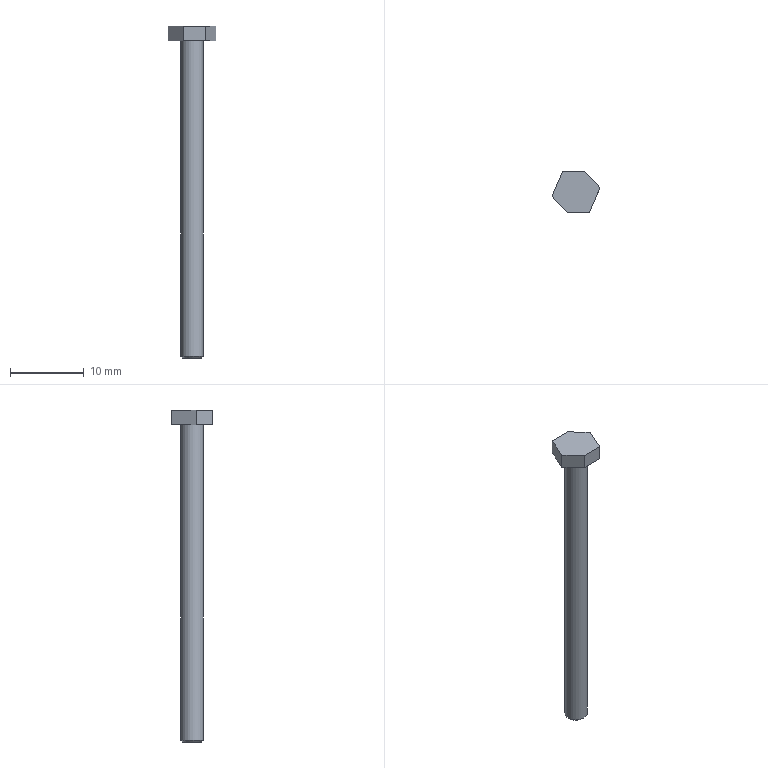Component | NX | LONG_SCREW_M3_2 | 1 solid | 11 faces | box 6.48 x 5.5 x 45 mm | volume 356 mm3 | plane 9 | cylinder 1 | cone 1 | commonest cylinder face diameters 3 x1
STEP:
#1=CARTESIAN_POINT('',(0.,0.,0.));
#2=DIRECTION('',(0.,0.,1.));
#3=DIRECTION('',(1.,0.,0.));
#4=AXIS2_PLACEMENT_3D('',#1,#2,#3);
#5=CARTESIAN_POINT('',(-13.131,-4.443,15.25));
#6=VERTEX_POINT('',#5);
#7=CARTESIAN_POINT('',(-14.506,-3.843,15.25));
#8=DIRECTION('',(0.,0.,1.));
#9=DIRECTION('',(0.9167,-0.3997,0.));
#10=AXIS2_PLACEMENT_3D('',#7,#8,#9);
#11=CIRCLE('',#10,1.5);
#12=CARTESIAN_POINT('',(-14.506,-3.843,15.));
#13=DIRECTION('',(0.,0.,1.));
#14=DIRECTION('',(0.9167,-0.3997,0.));
#15=AXIS2_PLACEMENT_3D('',#12,#13,#14);
#16=CYLINDRICAL_SURFACE('',#15,1.5);
#17=CARTESIAN_POINT('',(0.,0.25));
#18=DIRECTION('',(1.,0.));
#19=VECTOR('',#18,1.);
#20=LINE('',#17,#19);
#21=(GEOMETRIC_REPRESENTATION_CONTEXT(2)PARAMETRIC_REPRESENTATION_CONTEXT()REPRESENTATION_CONTEXT('',''));
#22=DEFINITIONAL_REPRESENTATION('',(#20),#21);
#23=PCURVE('',#16,#22);
#24=CARTESIAN_POINT('',(-14.506,-3.843,15.25));
#25=DIRECTION('',(0.,0.,1.));
#26=DIRECTION('',(0.9167,-0.3997,0.));
#27=AXIS2_PLACEMENT_3D('',#24,#25,#26);
#28=CONICAL_SURFACE('',#27,1.5,0.7854);
#29=CARTESIAN_POINT('',(0.,0.));
#30=DIRECTION('',(1.,0.));
#31=VECTOR('',#30,1.);
#32=LINE('',#29,#31);
#33=(GEOMETRIC_REPRESENTATION_CONTEXT(2)PARAMETRIC_REPRESENTATION_CONTEXT()REPRESENTATION_CONTEXT('',''));
#34=DEFINITIONAL_REPRESENTATION('',(#32),#33);
#35=PCURVE('',#28,#34);
#36=SURFACE_CURVE('',#11,(#23,#35),.PCURVE_S1.);
#37=EDGE_CURVE('',#6,#6,#36,.T.);
#38=ORIENTED_EDGE('',*,*,#37,.T.);
#39=CARTESIAN_POINT('',(-13.131,-4.443,58.));
#40=VERTEX_POINT('',#39);
#41=CARTESIAN_POINT('',(-13.131,-4.443,15.25));
#42=CARTESIAN_POINT('',(-13.131,-4.443,58.));
#43=B_SPLINE_CURVE_WITH_KNOTS('',1,(#41,#42),.UNSPECIFIED.,.F.,.F.,(2,2),(0.25,43.),.PIECEWISE_BEZIER_KNOTS.);
#44=CARTESIAN_POINT('',(6.283,0.));
#45=DIRECTION('',(0.,1.));
#46=VECTOR('',#45,1.);
#47=LINE('',#44,#46);
#48=(GEOMETRIC_REPRESENTATION_CONTEXT(2)PARAMETRIC_REPRESENTATION_CONTEXT()REPRESENTATION_CONTEXT('',''));
#49=DEFINITIONAL_REPRESENTATION('',(#47),#48);
#50=PCURVE('',#16,#49);
#51=CARTESIAN_POINT('',(0.,0.));
#52=DIRECTION('',(0.,1.));
#53=VECTOR('',#52,1.);
#54=LINE('',#51,#53);
#55=(GEOMETRIC_REPRESENTATION_CONTEXT(2)PARAMETRIC_REPRESENTATION_CONTEXT()REPRESENTATION_CONTEXT('',''));
#56=DEFINITIONAL_REPRESENTATION('',(#54),#55);
#57=PCURVE('',#16,#56);
#58=SEAM_CURVE('',#43,(#50,#57),.PCURVE_S1.);
#59=EDGE_CURVE('',#6,#40,#58,.T.);
#60=ORIENTED_EDGE('',*,*,#59,.T.);
#61=CARTESIAN_POINT('',(-14.506,-3.843,58.));
#62=DIRECTION('',(0.,0.,1.));
#63=DIRECTION('',(0.9167,-0.3997,0.));
#64=AXIS2_PLACEMENT_3D('',#61,#62,#63);
#65=CIRCLE('',#64,1.5);
#66=CARTESIAN_POINT('',(0.,43.));
#67=DIRECTION('',(1.,0.));
#68=VECTOR('',#67,1.);
#69=LINE('',#66,#68);
#70=(GEOMETRIC_REPRESENTATION_CONTEXT(2)PARAMETRIC_REPRESENTATION_CONTEXT()REPRESENTATION_CONTEXT('',''));
#71=DEFINITIONAL_REPRESENTATION('',(#69),#70);
#72=PCURVE('',#16,#71);
#73=CARTESIAN_POINT('',(-17.746,-4.395,58.));
#74=DIRECTION('',(0.,0.,1.));
#75=DIRECTION('',(0.9167,-0.3997,0.));
#76=AXIS2_PLACEMENT_3D('',#73,#74,#75);
#77=PLANE('',#76);
#78=CARTESIAN_POINT('',(2.75,1.801));
#79=DIRECTION('',(1.,-0.));
#80=AXIS2_PLACEMENT_2D('',#78,#79);
#81=CIRCLE('',#80,1.5);
#82=(GEOMETRIC_REPRESENTATION_CONTEXT(2)PARAMETRIC_REPRESENTATION_CONTEXT()REPRESENTATION_CONTEXT('',''));
#83=DEFINITIONAL_REPRESENTATION('',(#81),#82);
#84=PCURVE('',#77,#83);
#85=SURFACE_CURVE('',#65,(#72,#84),.PCURVE_S1.);
#86=EDGE_CURVE('',#40,#40,#85,.T.);
#87=ORIENTED_EDGE('',*,*,#86,.F.);
#88=ORIENTED_EDGE('',*,*,#59,.F.);
#89=EDGE_LOOP('',(#38,#60,#87,#88));
#90=FACE_BOUND('',#89,.T.);
#91=ADVANCED_FACE('',(#90),#16,.T.);
#92=CARTESIAN_POINT('',(-13.36,-4.343,15.));
#93=VERTEX_POINT('',#92);
#94=CARTESIAN_POINT('',(-14.506,-3.843,15.));
#95=DIRECTION('',(0.,0.,-1.));
#96=DIRECTION('',(0.9167,-0.3997,0.));
#97=AXIS2_PLACEMENT_3D('',#94,#95,#96);
#98=CIRCLE('',#97,1.25);
#99=CARTESIAN_POINT('',(-14.506,-3.843,15.));
#100=DIRECTION('',(0.,0.,1.));
#101=DIRECTION('',(0.9167,-0.3997,0.));
#102=AXIS2_PLACEMENT_3D('',#99,#100,#101);
#103=PLANE('',#102);
#104=CARTESIAN_POINT('',(1.25,0.));
#105=CARTESIAN_POINT('',(1.25,-2.165));
#106=CARTESIAN_POINT('',(-0.625,-1.083));
#107=CARTESIAN_POINT('',(-2.5,-0.));
#108=CARTESIAN_POINT('',(-0.625,1.083));
#109=CARTESIAN_POINT('',(1.25,2.165));
#110=CARTESIAN_POINT('',(1.25,0.));
#111=(BOUNDED_CURVE()B_SPLINE_CURVE(2,(#104,#105,#106,#107,#108,#109,#110),.UNSPECIFIED.,.T.,.F.)B_SPLINE_CURVE_WITH_KNOTS((1,2,2,2,2,1),(-2.094,0.,2.094,4.189,6.283,8.378),.UNSPECIFIED.)CURVE()GEOMETRIC_REPRESENTATION_ITEM()RATIONAL_B_SPLINE_CURVE((1.,0.5,1.,0.5,1.,0.5,1.))REPRESENTATION_ITEM(''));
#112=(GEOMETRIC_REPRESENTATION_CONTEXT(2)PARAMETRIC_REPRESENTATION_CONTEXT()REPRESENTATION_CONTEXT('',''));
#113=DEFINITIONAL_REPRESENTATION('',(#111),#112);
#114=PCURVE('',#103,#113);
#115=CARTESIAN_POINT('',(6.283,-0.25));
#116=DIRECTION('',(-1.,0.));
#117=VECTOR('',#116,1.);
#118=LINE('',#115,#117);
#119=(GEOMETRIC_REPRESENTATION_CONTEXT(2)PARAMETRIC_REPRESENTATION_CONTEXT()REPRESENTATION_CONTEXT('',''));
#120=DEFINITIONAL_REPRESENTATION('',(#118),#119);
#121=PCURVE('',#28,#120);
#122=SURFACE_CURVE('',#98,(#114,#121),.PCURVE_S1.);
#123=EDGE_CURVE('',#93,#93,#122,.T.);
#124=ORIENTED_EDGE('',*,*,#123,.T.);
#125=EDGE_LOOP('',(#124));
#126=FACE_BOUND('',#125,.T.);
#127=ADVANCED_FACE('',(#126),#103,.F.);
#128=CARTESIAN_POINT('',(-17.746,-4.395,58.));
#129=VERTEX_POINT('',#128);
#130=CARTESIAN_POINT('',(-15.705,-6.593,58.));
#131=VERTEX_POINT('',#130);
#132=CARTESIAN_POINT('',(-17.746,-4.395,58.));
#133=DIRECTION('',(0.6806,-0.7327,0.));
#134=VECTOR('',#133,1.);
#135=LINE('',#132,#134);
#136=CARTESIAN_POINT('',(0.,0.));
#137=DIRECTION('',(0.9167,-0.3997));
#138=VECTOR('',#137,1.);
#139=LINE('',#136,#138);
#140=(GEOMETRIC_REPRESENTATION_CONTEXT(2)PARAMETRIC_REPRESENTATION_CONTEXT()REPRESENTATION_CONTEXT('',''));
#141=DEFINITIONAL_REPRESENTATION('',(#139),#140);
#142=PCURVE('',#77,#141);
#143=CARTESIAN_POINT('',(-17.746,-4.395,60.));
#144=DIRECTION('',(0.7327,0.6806,0.));
#145=DIRECTION('',(-0.6806,0.7327,0.));
#146=AXIS2_PLACEMENT_3D('',#143,#144,#145);
#147=PLANE('',#146);
#148=CARTESIAN_POINT('',(0.,-2.));
#149=DIRECTION('',(-1.,0.));
#150=VECTOR('',#149,1.);
#151=LINE('',#148,#150);
#152=(GEOMETRIC_REPRESENTATION_CONTEXT(2)PARAMETRIC_REPRESENTATION_CONTEXT()REPRESENTATION_CONTEXT('',''));
#153=DEFINITIONAL_REPRESENTATION('',(#151),#152);
#154=PCURVE('',#147,#153);
#155=SURFACE_CURVE('',#135,(#142,#154),.PCURVE_S1.);
#156=EDGE_CURVE('',#129,#131,#155,.T.);
#157=ORIENTED_EDGE('',*,*,#156,.F.);
#158=CARTESIAN_POINT('',(-16.307,-1.093,58.));
#159=VERTEX_POINT('',#158);
#160=CARTESIAN_POINT('',(-16.307,-1.093,58.));
#161=DIRECTION('',(-0.3997,-0.9167,0.));
#162=VECTOR('',#161,1.);
#163=LINE('',#160,#162);
#164=CARTESIAN_POINT('',(0.,3.602));
#165=DIRECTION('',(-0.,-1.));
#166=VECTOR('',#165,1.);
#167=LINE('',#164,#166);
#168=(GEOMETRIC_REPRESENTATION_CONTEXT(2)PARAMETRIC_REPRESENTATION_CONTEXT()REPRESENTATION_CONTEXT('',''));
#169=DEFINITIONAL_REPRESENTATION('',(#167),#168);
#170=PCURVE('',#77,#169);
#171=CARTESIAN_POINT('',(-16.307,-1.093,60.));
#172=DIRECTION('',(0.9167,-0.3997,0.));
#173=DIRECTION('',(0.3997,0.9167,0.));
#174=AXIS2_PLACEMENT_3D('',#171,#172,#173);
#175=PLANE('',#174);
#176=CARTESIAN_POINT('',(0.,-2.));
#177=DIRECTION('',(-1.,0.));
#178=VECTOR('',#177,1.);
#179=LINE('',#176,#178);
#180=(GEOMETRIC_REPRESENTATION_CONTEXT(2)PARAMETRIC_REPRESENTATION_CONTEXT()REPRESENTATION_CONTEXT('',''));
#181=DEFINITIONAL_REPRESENTATION('',(#179),#180);
#182=PCURVE('',#175,#181);
#183=SURFACE_CURVE('',#163,(#170,#182),.PCURVE_S1.);
#184=EDGE_CURVE('',#159,#129,#183,.T.);
#185=ORIENTED_EDGE('',*,*,#184,.F.);
#186=CARTESIAN_POINT('',(-13.307,-1.093,58.));
#187=VERTEX_POINT('',#186);
#188=CARTESIAN_POINT('',(-13.307,-1.093,58.));
#189=DIRECTION('',(-1.,0.,0.));
#190=VECTOR('',#189,1.);
#191=LINE('',#188,#190);
#192=CARTESIAN_POINT('',(2.75,4.801));
#193=DIRECTION('',(-0.9167,-0.3997));
#194=VECTOR('',#193,1.);
#195=LINE('',#192,#194);
#196=(GEOMETRIC_REPRESENTATION_CONTEXT(2)PARAMETRIC_REPRESENTATION_CONTEXT()REPRESENTATION_CONTEXT('',''));
#197=DEFINITIONAL_REPRESENTATION('',(#195),#196);
#198=PCURVE('',#77,#197);
#199=CARTESIAN_POINT('',(-13.307,-1.093,60.));
#200=DIRECTION('',(-0.,-1.,0.));
#201=DIRECTION('',(1.,-0.,0.));
#202=AXIS2_PLACEMENT_3D('',#199,#200,#201);
#203=PLANE('',#202);
#204=CARTESIAN_POINT('',(0.,-2.));
#205=DIRECTION('',(-1.,0.));
#206=VECTOR('',#205,1.);
#207=LINE('',#204,#206);
#208=(GEOMETRIC_REPRESENTATION_CONTEXT(2)PARAMETRIC_REPRESENTATION_CONTEXT()REPRESENTATION_CONTEXT('',''));
#209=DEFINITIONAL_REPRESENTATION('',(#207),#208);
#210=PCURVE('',#203,#209);
#211=SURFACE_CURVE('',#191,(#198,#210),.PCURVE_S1.);
#212=EDGE_CURVE('',#187,#159,#211,.T.);
#213=ORIENTED_EDGE('',*,*,#212,.F.);
#214=CARTESIAN_POINT('',(-11.265,-3.291,58.));
#215=VERTEX_POINT('',#214);
#216=CARTESIAN_POINT('',(-11.265,-3.291,58.));
#217=DIRECTION('',(-0.6806,0.7327,0.));
#218=VECTOR('',#217,1.);
#219=LINE('',#216,#218);
#220=CARTESIAN_POINT('',(5.5,3.602));
#221=DIRECTION('',(-0.9167,0.3997));
#222=VECTOR('',#221,1.);
#223=LINE('',#220,#222);
#224=(GEOMETRIC_REPRESENTATION_CONTEXT(2)PARAMETRIC_REPRESENTATION_CONTEXT()REPRESENTATION_CONTEXT('',''));
#225=DEFINITIONAL_REPRESENTATION('',(#223),#224);
#226=PCURVE('',#77,#225);
#227=CARTESIAN_POINT('',(-11.265,-3.291,60.));
#228=DIRECTION('',(-0.7327,-0.6806,0.));
#229=DIRECTION('',(0.6806,-0.7327,0.));
#230=AXIS2_PLACEMENT_3D('',#227,#228,#229);
#231=PLANE('',#230);
#232=CARTESIAN_POINT('',(0.,-2.));
#233=DIRECTION('',(-1.,0.));
#234=VECTOR('',#233,1.);
#235=LINE('',#232,#234);
#236=(GEOMETRIC_REPRESENTATION_CONTEXT(2)PARAMETRIC_REPRESENTATION_CONTEXT()REPRESENTATION_CONTEXT('',''));
#237=DEFINITIONAL_REPRESENTATION('',(#235),#236);
#238=PCURVE('',#231,#237);
#239=SURFACE_CURVE('',#219,(#226,#238),.PCURVE_S1.);
#240=EDGE_CURVE('',#215,#187,#239,.T.);
#241=ORIENTED_EDGE('',*,*,#240,.F.);
#242=CARTESIAN_POINT('',(-12.705,-6.593,58.));
#243=VERTEX_POINT('',#242);
#244=CARTESIAN_POINT('',(-11.985,-4.942,58.));
#245=DIRECTION('',(0.3997,0.9167,0.));
#246=VECTOR('',#245,1.);
#247=LINE('',#244,#246);
#248=CARTESIAN_POINT('',(5.5,1.801));
#249=DIRECTION('',(0.,1.));
#250=VECTOR('',#249,1.);
#251=LINE('',#248,#250);
#252=(GEOMETRIC_REPRESENTATION_CONTEXT(2)PARAMETRIC_REPRESENTATION_CONTEXT()REPRESENTATION_CONTEXT('',''));
#253=DEFINITIONAL_REPRESENTATION('',(#251),#252);
#254=PCURVE('',#77,#253);
#255=CARTESIAN_POINT('',(-11.985,-4.942,60.));
#256=DIRECTION('',(-0.9167,0.3997,0.));
#257=DIRECTION('',(0.,0.,1.));
#258=AXIS2_PLACEMENT_3D('',#255,#256,#257);
#259=PLANE('',#258);
#260=CARTESIAN_POINT('',(-2.,0.));
#261=DIRECTION('',(0.,1.));
#262=VECTOR('',#261,1.);
#263=LINE('',#260,#262);
#264=(GEOMETRIC_REPRESENTATION_CONTEXT(2)PARAMETRIC_REPRESENTATION_CONTEXT()REPRESENTATION_CONTEXT('',''));
#265=DEFINITIONAL_REPRESENTATION('',(#263),#264);
#266=PCURVE('',#259,#265);
#267=SURFACE_CURVE('',#247,(#254,#266),.PCURVE_S1.);
#268=EDGE_CURVE('',#243,#215,#267,.T.);
#269=ORIENTED_EDGE('',*,*,#268,.F.);
#270=CARTESIAN_POINT('',(-15.705,-6.593,58.));
#271=DIRECTION('',(1.,0.,0.));
#272=VECTOR('',#271,1.);
#273=LINE('',#270,#272);
#274=CARTESIAN_POINT('',(2.75,-1.199));
#275=DIRECTION('',(0.9167,0.3997));
#276=VECTOR('',#275,1.);
#277=LINE('',#274,#276);
#278=(GEOMETRIC_REPRESENTATION_CONTEXT(2)PARAMETRIC_REPRESENTATION_CONTEXT()REPRESENTATION_CONTEXT('',''));
#279=DEFINITIONAL_REPRESENTATION('',(#277),#278);
#280=PCURVE('',#77,#279);
#281=CARTESIAN_POINT('',(-15.705,-6.593,60.));
#282=DIRECTION('',(0.,1.,0.));
#283=DIRECTION('',(-1.,0.,0.));
#284=AXIS2_PLACEMENT_3D('',#281,#282,#283);
#285=PLANE('',#284);
#286=CARTESIAN_POINT('',(0.,-2.));
#287=DIRECTION('',(-1.,0.));
#288=VECTOR('',#287,1.);
#289=LINE('',#286,#288);
#290=(GEOMETRIC_REPRESENTATION_CONTEXT(2)PARAMETRIC_REPRESENTATION_CONTEXT()REPRESENTATION_CONTEXT('',''));
#291=DEFINITIONAL_REPRESENTATION('',(#289),#290);
#292=PCURVE('',#285,#291);
#293=SURFACE_CURVE('',#273,(#280,#292),.PCURVE_S1.);
#294=EDGE_CURVE('',#131,#243,#293,.T.);
#295=ORIENTED_EDGE('',*,*,#294,.F.);
#296=EDGE_LOOP('',(#157,#185,#213,#241,#269,#295));
#297=FACE_BOUND('',#296,.T.);
#298=ORIENTED_EDGE('',*,*,#86,.T.);
#299=EDGE_LOOP('',(#298));
#300=FACE_BOUND('',#299,.T.);
#301=ADVANCED_FACE('',(#297,#300),#77,.F.);
#302=ORIENTED_EDGE('',*,*,#156,.T.);
#303=CARTESIAN_POINT('',(-15.705,-6.593,60.));
#304=VERTEX_POINT('',#303);
#305=CARTESIAN_POINT('',(-15.705,-6.593,60.));
#306=DIRECTION('',(0.,0.,-1.));
#307=VECTOR('',#306,1.);
#308=LINE('',#305,#307);
#309=CARTESIAN_POINT('',(-3.,0.));
#310=DIRECTION('',(0.,-1.));
#311=VECTOR('',#310,1.);
#312=LINE('',#309,#311);
#313=(GEOMETRIC_REPRESENTATION_CONTEXT(2)PARAMETRIC_REPRESENTATION_CONTEXT()REPRESENTATION_CONTEXT('',''));
#314=DEFINITIONAL_REPRESENTATION('',(#312),#313);
#315=PCURVE('',#147,#314);
#316=CARTESIAN_POINT('',(0.,0.));
#317=DIRECTION('',(0.,-1.));
#318=VECTOR('',#317,1.);
#319=LINE('',#316,#318);
#320=(GEOMETRIC_REPRESENTATION_CONTEXT(2)PARAMETRIC_REPRESENTATION_CONTEXT()REPRESENTATION_CONTEXT('',''));
#321=DEFINITIONAL_REPRESENTATION('',(#319),#320);
#322=PCURVE('',#285,#321);
#323=SURFACE_CURVE('',#308,(#315,#322),.PCURVE_S1.);
#324=EDGE_CURVE('',#304,#131,#323,.T.);
#325=ORIENTED_EDGE('',*,*,#324,.F.);
#326=CARTESIAN_POINT('',(-17.746,-4.395,60.));
#327=VERTEX_POINT('',#326);
#328=CARTESIAN_POINT('',(-17.746,-4.395,60.));
#329=DIRECTION('',(0.6806,-0.7327,0.));
#330=VECTOR('',#329,1.);
#331=LINE('',#328,#330);
#332=CARTESIAN_POINT('',(0.,0.));
#333=DIRECTION('',(-1.,0.));
#334=VECTOR('',#333,1.);
#335=LINE('',#332,#334);
#336=(GEOMETRIC_REPRESENTATION_CONTEXT(2)PARAMETRIC_REPRESENTATION_CONTEXT()REPRESENTATION_CONTEXT('',''));
#337=DEFINITIONAL_REPRESENTATION('',(#335),#336);
#338=PCURVE('',#147,#337);
#339=CARTESIAN_POINT('',(-17.746,-4.395,60.));
#340=DIRECTION('',(0.,0.,1.));
#341=DIRECTION('',(0.9167,-0.3997,0.));
#342=AXIS2_PLACEMENT_3D('',#339,#340,#341);
#343=PLANE('',#342);
#344=CARTESIAN_POINT('',(0.,0.));
#345=DIRECTION('',(0.9167,-0.3997));
#346=VECTOR('',#345,1.);
#347=LINE('',#344,#346);
#348=(GEOMETRIC_REPRESENTATION_CONTEXT(2)PARAMETRIC_REPRESENTATION_CONTEXT()REPRESENTATION_CONTEXT('',''));
#349=DEFINITIONAL_REPRESENTATION('',(#347),#348);
#350=PCURVE('',#343,#349);
#351=SURFACE_CURVE('',#331,(#338,#350),.PCURVE_S1.);
#352=EDGE_CURVE('',#327,#304,#351,.T.);
#353=ORIENTED_EDGE('',*,*,#352,.F.);
#354=CARTESIAN_POINT('',(-17.746,-4.395,60.));
#355=DIRECTION('',(0.,0.,-1.));
#356=VECTOR('',#355,1.);
#357=LINE('',#354,#356);
#358=CARTESIAN_POINT('',(0.,0.));
#359=DIRECTION('',(0.,-1.));
#360=VECTOR('',#359,1.);
#361=LINE('',#358,#360);
#362=(GEOMETRIC_REPRESENTATION_CONTEXT(2)PARAMETRIC_REPRESENTATION_CONTEXT()REPRESENTATION_CONTEXT('',''));
#363=DEFINITIONAL_REPRESENTATION('',(#361),#362);
#364=PCURVE('',#147,#363);
#365=CARTESIAN_POINT('',(-3.602,0.));
#366=DIRECTION('',(0.,-1.));
#367=VECTOR('',#366,1.);
#368=LINE('',#365,#367);
#369=(GEOMETRIC_REPRESENTATION_CONTEXT(2)PARAMETRIC_REPRESENTATION_CONTEXT()REPRESENTATION_CONTEXT('',''));
#370=DEFINITIONAL_REPRESENTATION('',(#368),#369);
#371=PCURVE('',#175,#370);
#372=SURFACE_CURVE('',#357,(#364,#371),.PCURVE_S1.);
#373=EDGE_CURVE('',#327,#129,#372,.T.);
#374=ORIENTED_EDGE('',*,*,#373,.T.);
#375=EDGE_LOOP('',(#302,#325,#353,#374));
#376=FACE_BOUND('',#375,.T.);
#377=ADVANCED_FACE('',(#376),#147,.F.);
#378=ORIENTED_EDGE('',*,*,#294,.T.);
#379=CARTESIAN_POINT('',(-12.705,-6.593,60.));
#380=VERTEX_POINT('',#379);
#381=CARTESIAN_POINT('',(-12.705,-6.593,60.));
#382=DIRECTION('',(0.,0.,-1.));
#383=VECTOR('',#382,1.);
#384=LINE('',#381,#383);
#385=CARTESIAN_POINT('',(-3.,0.));
#386=DIRECTION('',(0.,-1.));
#387=VECTOR('',#386,1.);
#388=LINE('',#385,#387);
#389=(GEOMETRIC_REPRESENTATION_CONTEXT(2)PARAMETRIC_REPRESENTATION_CONTEXT()REPRESENTATION_CONTEXT('',''));
#390=DEFINITIONAL_REPRESENTATION('',(#388),#389);
#391=PCURVE('',#285,#390);
#392=CARTESIAN_POINT('',(0.,-1.801));
#393=DIRECTION('',(-1.,0.));
#394=VECTOR('',#393,1.);
#395=LINE('',#392,#394);
#396=(GEOMETRIC_REPRESENTATION_CONTEXT(2)PARAMETRIC_REPRESENTATION_CONTEXT()REPRESENTATION_CONTEXT('',''));
#397=DEFINITIONAL_REPRESENTATION('',(#395),#396);
#398=PCURVE('',#259,#397);
#399=SURFACE_CURVE('',#384,(#391,#398),.PCURVE_S1.);
#400=EDGE_CURVE('',#380,#243,#399,.T.);
#401=ORIENTED_EDGE('',*,*,#400,.F.);
#402=CARTESIAN_POINT('',(-15.705,-6.593,60.));
#403=DIRECTION('',(1.,0.,0.));
#404=VECTOR('',#403,1.);
#405=LINE('',#402,#404);
#406=CARTESIAN_POINT('',(0.,0.));
#407=DIRECTION('',(-1.,0.));
#408=VECTOR('',#407,1.);
#409=LINE('',#406,#408);
#410=(GEOMETRIC_REPRESENTATION_CONTEXT(2)PARAMETRIC_REPRESENTATION_CONTEXT()REPRESENTATION_CONTEXT('',''));
#411=DEFINITIONAL_REPRESENTATION('',(#409),#410);
#412=PCURVE('',#285,#411);
#413=CARTESIAN_POINT('',(2.75,-1.199));
#414=DIRECTION('',(0.9167,0.3997));
#415=VECTOR('',#414,1.);
#416=LINE('',#413,#415);
#417=(GEOMETRIC_REPRESENTATION_CONTEXT(2)PARAMETRIC_REPRESENTATION_CONTEXT()REPRESENTATION_CONTEXT('',''));
#418=DEFINITIONAL_REPRESENTATION('',(#416),#417);
#419=PCURVE('',#343,#418);
#420=SURFACE_CURVE('',#405,(#412,#419),.PCURVE_S1.);
#421=EDGE_CURVE('',#304,#380,#420,.T.);
#422=ORIENTED_EDGE('',*,*,#421,.F.);
#423=ORIENTED_EDGE('',*,*,#324,.T.);
#424=EDGE_LOOP('',(#378,#401,#422,#423));
#425=FACE_BOUND('',#424,.T.);
#426=ADVANCED_FACE('',(#425),#285,.F.);
#427=ORIENTED_EDGE('',*,*,#268,.T.);
#428=CARTESIAN_POINT('',(-11.265,-3.291,60.));
#429=VERTEX_POINT('',#428);
#430=CARTESIAN_POINT('',(-11.265,-3.291,60.));
#431=DIRECTION('',(0.,0.,-1.));
#432=VECTOR('',#431,1.);
#433=LINE('',#430,#432);
#434=CARTESIAN_POINT('',(0.,1.801));
#435=DIRECTION('',(-1.,0.));
#436=VECTOR('',#435,1.);
#437=LINE('',#434,#436);
#438=(GEOMETRIC_REPRESENTATION_CONTEXT(2)PARAMETRIC_REPRESENTATION_CONTEXT()REPRESENTATION_CONTEXT('',''));
#439=DEFINITIONAL_REPRESENTATION('',(#437),#438);
#440=PCURVE('',#259,#439);
#441=CARTESIAN_POINT('',(0.,0.));
#442=DIRECTION('',(0.,-1.));
#443=VECTOR('',#442,1.);
#444=LINE('',#441,#443);
#445=(GEOMETRIC_REPRESENTATION_CONTEXT(2)PARAMETRIC_REPRESENTATION_CONTEXT()REPRESENTATION_CONTEXT('',''));
#446=DEFINITIONAL_REPRESENTATION('',(#444),#445);
#447=PCURVE('',#231,#446);
#448=SURFACE_CURVE('',#433,(#440,#447),.PCURVE_S1.);
#449=EDGE_CURVE('',#429,#215,#448,.T.);
#450=ORIENTED_EDGE('',*,*,#449,.F.);
#451=CARTESIAN_POINT('',(-12.705,-6.593,60.));
#452=DIRECTION('',(0.3997,0.9167,0.));
#453=VECTOR('',#452,1.);
#454=LINE('',#451,#453);
#455=CARTESIAN_POINT('',(0.,-1.801));
#456=DIRECTION('',(0.,1.));
#457=VECTOR('',#456,1.);
#458=LINE('',#455,#457);
#459=(GEOMETRIC_REPRESENTATION_CONTEXT(2)PARAMETRIC_REPRESENTATION_CONTEXT()REPRESENTATION_CONTEXT('',''));
#460=DEFINITIONAL_REPRESENTATION('',(#458),#459);
#461=PCURVE('',#259,#460);
#462=CARTESIAN_POINT('',(5.5,0.));
#463=DIRECTION('',(0.,1.));
#464=VECTOR('',#463,1.);
#465=LINE('',#462,#464);
#466=(GEOMETRIC_REPRESENTATION_CONTEXT(2)PARAMETRIC_REPRESENTATION_CONTEXT()REPRESENTATION_CONTEXT('',''));
#467=DEFINITIONAL_REPRESENTATION('',(#465),#466);
#468=PCURVE('',#343,#467);
#469=SURFACE_CURVE('',#454,(#461,#468),.PCURVE_S1.);
#470=EDGE_CURVE('',#380,#429,#469,.T.);
#471=ORIENTED_EDGE('',*,*,#470,.F.);
#472=ORIENTED_EDGE('',*,*,#400,.T.);
#473=EDGE_LOOP('',(#427,#450,#471,#472));
#474=FACE_BOUND('',#473,.T.);
#475=ADVANCED_FACE('',(#474),#259,.F.);
#476=ORIENTED_EDGE('',*,*,#240,.T.);
#477=CARTESIAN_POINT('',(-13.307,-1.093,60.));
#478=VERTEX_POINT('',#477);
#479=CARTESIAN_POINT('',(-13.307,-1.093,60.));
#480=DIRECTION('',(0.,0.,-1.));
#481=VECTOR('',#480,1.);
#482=LINE('',#479,#481);
#483=CARTESIAN_POINT('',(-3.,0.));
#484=DIRECTION('',(0.,-1.));
#485=VECTOR('',#484,1.);
#486=LINE('',#483,#485);
#487=(GEOMETRIC_REPRESENTATION_CONTEXT(2)PARAMETRIC_REPRESENTATION_CONTEXT()REPRESENTATION_CONTEXT('',''));
#488=DEFINITIONAL_REPRESENTATION('',(#486),#487);
#489=PCURVE('',#231,#488);
#490=CARTESIAN_POINT('',(0.,0.));
#491=DIRECTION('',(0.,-1.));
#492=VECTOR('',#491,1.);
#493=LINE('',#490,#492);
#494=(GEOMETRIC_REPRESENTATION_CONTEXT(2)PARAMETRIC_REPRESENTATION_CONTEXT()REPRESENTATION_CONTEXT('',''));
#495=DEFINITIONAL_REPRESENTATION('',(#493),#494);
#496=PCURVE('',#203,#495);
#497=SURFACE_CURVE('',#482,(#489,#496),.PCURVE_S1.);
#498=EDGE_CURVE('',#478,#187,#497,.T.);
#499=ORIENTED_EDGE('',*,*,#498,.F.);
#500=CARTESIAN_POINT('',(-11.265,-3.291,60.));
#501=DIRECTION('',(-0.6806,0.7327,0.));
#502=VECTOR('',#501,1.);
#503=LINE('',#500,#502);
#504=CARTESIAN_POINT('',(0.,0.));
#505=DIRECTION('',(-1.,0.));
#506=VECTOR('',#505,1.);
#507=LINE('',#504,#506);
#508=(GEOMETRIC_REPRESENTATION_CONTEXT(2)PARAMETRIC_REPRESENTATION_CONTEXT()REPRESENTATION_CONTEXT('',''));
#509=DEFINITIONAL_REPRESENTATION('',(#507),#508);
#510=PCURVE('',#231,#509);
#511=CARTESIAN_POINT('',(5.5,3.602));
#512=DIRECTION('',(-0.9167,0.3997));
#513=VECTOR('',#512,1.);
#514=LINE('',#511,#513);
#515=(GEOMETRIC_REPRESENTATION_CONTEXT(2)PARAMETRIC_REPRESENTATION_CONTEXT()REPRESENTATION_CONTEXT('',''));
#516=DEFINITIONAL_REPRESENTATION('',(#514),#515);
#517=PCURVE('',#343,#516);
#518=SURFACE_CURVE('',#503,(#510,#517),.PCURVE_S1.);
#519=EDGE_CURVE('',#429,#478,#518,.T.);
#520=ORIENTED_EDGE('',*,*,#519,.F.);
#521=ORIENTED_EDGE('',*,*,#449,.T.);
#522=EDGE_LOOP('',(#476,#499,#520,#521));
#523=FACE_BOUND('',#522,.T.);
#524=ADVANCED_FACE('',(#523),#231,.F.);
#525=ORIENTED_EDGE('',*,*,#212,.T.);
#526=CARTESIAN_POINT('',(-16.307,-1.093,60.));
#527=VERTEX_POINT('',#526);
#528=CARTESIAN_POINT('',(-16.307,-1.093,60.));
#529=DIRECTION('',(0.,0.,-1.));
#530=VECTOR('',#529,1.);
#531=LINE('',#528,#530);
#532=CARTESIAN_POINT('',(-3.,0.));
#533=DIRECTION('',(0.,-1.));
#534=VECTOR('',#533,1.);
#535=LINE('',#532,#534);
#536=(GEOMETRIC_REPRESENTATION_CONTEXT(2)PARAMETRIC_REPRESENTATION_CONTEXT()REPRESENTATION_CONTEXT('',''));
#537=DEFINITIONAL_REPRESENTATION('',(#535),#536);
#538=PCURVE('',#203,#537);
#539=CARTESIAN_POINT('',(0.,0.));
#540=DIRECTION('',(0.,-1.));
#541=VECTOR('',#540,1.);
#542=LINE('',#539,#541);
#543=(GEOMETRIC_REPRESENTATION_CONTEXT(2)PARAMETRIC_REPRESENTATION_CONTEXT()REPRESENTATION_CONTEXT('',''));
#544=DEFINITIONAL_REPRESENTATION('',(#542),#543);
#545=PCURVE('',#175,#544);
#546=SURFACE_CURVE('',#531,(#538,#545),.PCURVE_S1.);
#547=EDGE_CURVE('',#527,#159,#546,.T.);
#548=ORIENTED_EDGE('',*,*,#547,.F.);
#549=CARTESIAN_POINT('',(-13.307,-1.093,60.));
#550=DIRECTION('',(-1.,0.,0.));
#551=VECTOR('',#550,1.);
#552=LINE('',#549,#551);
#553=CARTESIAN_POINT('',(0.,0.));
#554=DIRECTION('',(-1.,0.));
#555=VECTOR('',#554,1.);
#556=LINE('',#553,#555);
#557=(GEOMETRIC_REPRESENTATION_CONTEXT(2)PARAMETRIC_REPRESENTATION_CONTEXT()REPRESENTATION_CONTEXT('',''));
#558=DEFINITIONAL_REPRESENTATION('',(#556),#557);
#559=PCURVE('',#203,#558);
#560=CARTESIAN_POINT('',(2.75,4.801));
#561=DIRECTION('',(-0.9167,-0.3997));
#562=VECTOR('',#561,1.);
#563=LINE('',#560,#562);
#564=(GEOMETRIC_REPRESENTATION_CONTEXT(2)PARAMETRIC_REPRESENTATION_CONTEXT()REPRESENTATION_CONTEXT('',''));
#565=DEFINITIONAL_REPRESENTATION('',(#563),#564);
#566=PCURVE('',#343,#565);
#567=SURFACE_CURVE('',#552,(#559,#566),.PCURVE_S1.);
#568=EDGE_CURVE('',#478,#527,#567,.T.);
#569=ORIENTED_EDGE('',*,*,#568,.F.);
#570=ORIENTED_EDGE('',*,*,#498,.T.);
#571=EDGE_LOOP('',(#525,#548,#569,#570));
#572=FACE_BOUND('',#571,.T.);
#573=ADVANCED_FACE('',(#572),#203,.F.);
#574=ORIENTED_EDGE('',*,*,#184,.T.);
#575=ORIENTED_EDGE('',*,*,#373,.F.);
#576=CARTESIAN_POINT('',(-17.026,-2.744,60.));
#577=DIRECTION('',(-0.3997,-0.9167,0.));
#578=VECTOR('',#577,1.);
#579=LINE('',#576,#578);
#580=CARTESIAN_POINT('',(-1.801,0.));
#581=DIRECTION('',(-1.,0.));
#582=VECTOR('',#581,1.);
#583=LINE('',#580,#582);
#584=(GEOMETRIC_REPRESENTATION_CONTEXT(2)PARAMETRIC_REPRESENTATION_CONTEXT()REPRESENTATION_CONTEXT('',''));
#585=DEFINITIONAL_REPRESENTATION('',(#583),#584);
#586=PCURVE('',#175,#585);
#587=CARTESIAN_POINT('',(0.,1.801));
#588=DIRECTION('',(0.,-1.));
#589=VECTOR('',#588,1.);
#590=LINE('',#587,#589);
#591=(GEOMETRIC_REPRESENTATION_CONTEXT(2)PARAMETRIC_REPRESENTATION_CONTEXT()REPRESENTATION_CONTEXT('',''));
#592=DEFINITIONAL_REPRESENTATION('',(#590),#591);
#593=PCURVE('',#343,#592);
#594=SURFACE_CURVE('',#579,(#586,#593),.PCURVE_S1.);
#595=EDGE_CURVE('',#527,#327,#594,.T.);
#596=ORIENTED_EDGE('',*,*,#595,.F.);
#597=ORIENTED_EDGE('',*,*,#547,.T.);
#598=EDGE_LOOP('',(#574,#575,#596,#597));
#599=FACE_BOUND('',#598,.T.);
#600=ADVANCED_FACE('',(#599),#175,.F.);
#601=ORIENTED_EDGE('',*,*,#595,.T.);
#602=ORIENTED_EDGE('',*,*,#352,.T.);
#603=ORIENTED_EDGE('',*,*,#421,.T.);
#604=ORIENTED_EDGE('',*,*,#470,.T.);
#605=ORIENTED_EDGE('',*,*,#519,.T.);
#606=ORIENTED_EDGE('',*,*,#568,.T.);
#607=EDGE_LOOP('',(#601,#602,#603,#604,#605,#606));
#608=FACE_BOUND('',#607,.T.);
#609=ADVANCED_FACE('',(#608),#343,.T.);
#610=ORIENTED_EDGE('',*,*,#123,.F.);
#611=CARTESIAN_POINT('',(-13.36,-4.343,15.));
#612=CARTESIAN_POINT('',(-13.131,-4.443,15.25));
#613=B_SPLINE_CURVE_WITH_KNOTS('',1,(#611,#612),.UNSPECIFIED.,.F.,.F.,(2,2),(-0.3536,0.),.PIECEWISE_BEZIER_KNOTS.);
#614=CARTESIAN_POINT('',(6.283,0.));
#615=DIRECTION('',(0.,1.));
#616=VECTOR('',#615,1.);
#617=LINE('',#614,#616);
#618=(GEOMETRIC_REPRESENTATION_CONTEXT(2)PARAMETRIC_REPRESENTATION_CONTEXT()REPRESENTATION_CONTEXT('',''));
#619=DEFINITIONAL_REPRESENTATION('',(#617),#618);
#620=PCURVE('',#28,#619);
#621=CARTESIAN_POINT('',(0.,0.));
#622=DIRECTION('',(0.,1.));
#623=VECTOR('',#622,1.);
#624=LINE('',#621,#623);
#625=(GEOMETRIC_REPRESENTATION_CONTEXT(2)PARAMETRIC_REPRESENTATION_CONTEXT()REPRESENTATION_CONTEXT('',''));
#626=DEFINITIONAL_REPRESENTATION('',(#624),#625);
#627=PCURVE('',#28,#626);
#628=SEAM_CURVE('',#613,(#620,#627),.PCURVE_S1.);
#629=EDGE_CURVE('',#93,#6,#628,.T.);
#630=ORIENTED_EDGE('',*,*,#629,.T.);
#631=ORIENTED_EDGE('',*,*,#37,.F.);
#632=ORIENTED_EDGE('',*,*,#629,.F.);
#633=EDGE_LOOP('',(#610,#630,#631,#632));
#634=FACE_BOUND('',#633,.T.);
#635=ADVANCED_FACE('',(#634),#28,.T.);
#636=CLOSED_SHELL('',(#91,#127,#301,#377,#426,#475,#524,#573,#600,#609,#635));
#637=MANIFOLD_SOLID_BREP('',#636);
#638=(LENGTH_UNIT()NAMED_UNIT(*)SI_UNIT(.MILLI.,.METRE.));
#639=UNCERTAINTY_MEASURE_WITH_UNIT(LENGTH_MEASURE(0.000002),#638,'','');
#640=(NAMED_UNIT(*)PLANE_ANGLE_UNIT()SI_UNIT($,.RADIAN.));
#641=(NAMED_UNIT(*)SI_UNIT($,.STERADIAN.)SOLID_ANGLE_UNIT());
#642=(GEOMETRIC_REPRESENTATION_CONTEXT(3)GLOBAL_UNCERTAINTY_ASSIGNED_CONTEXT((#639))GLOBAL_UNIT_ASSIGNED_CONTEXT((#638,#640,#641))REPRESENTATION_CONTEXT('',''));
#643=ADVANCED_BREP_SHAPE_REPRESENTATION('',(#4,#637),#642);